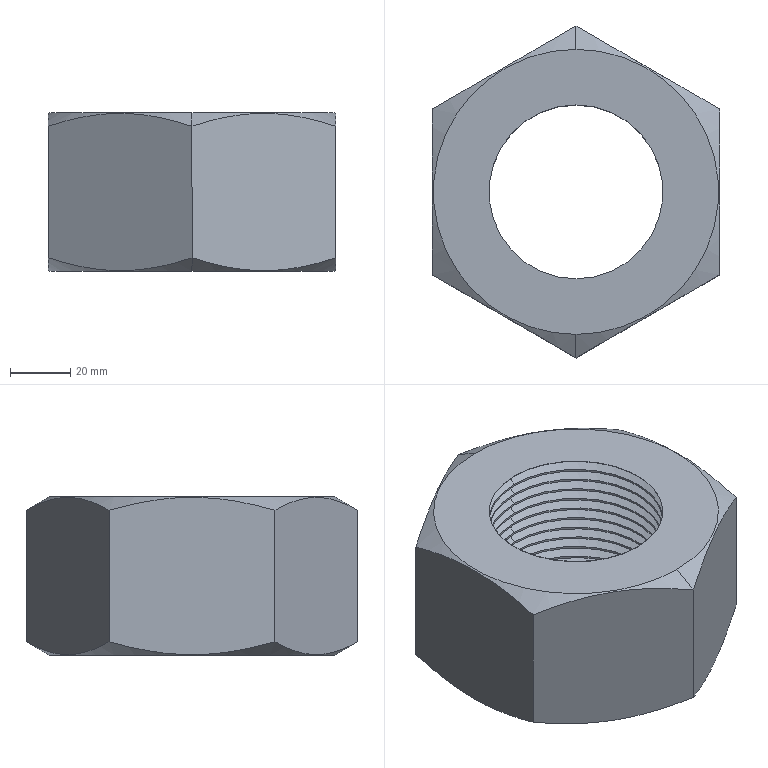Component | SolidWorks | TopPlate-1_TopPanelInnerPanel-2_hexagon nuts grade c gb-5 | 1 solid | 94 faces | volume 259759 mm3 | cone 58 | cylinder 28 | plane 8 | commonest cylinder face diameters 57.505 x28